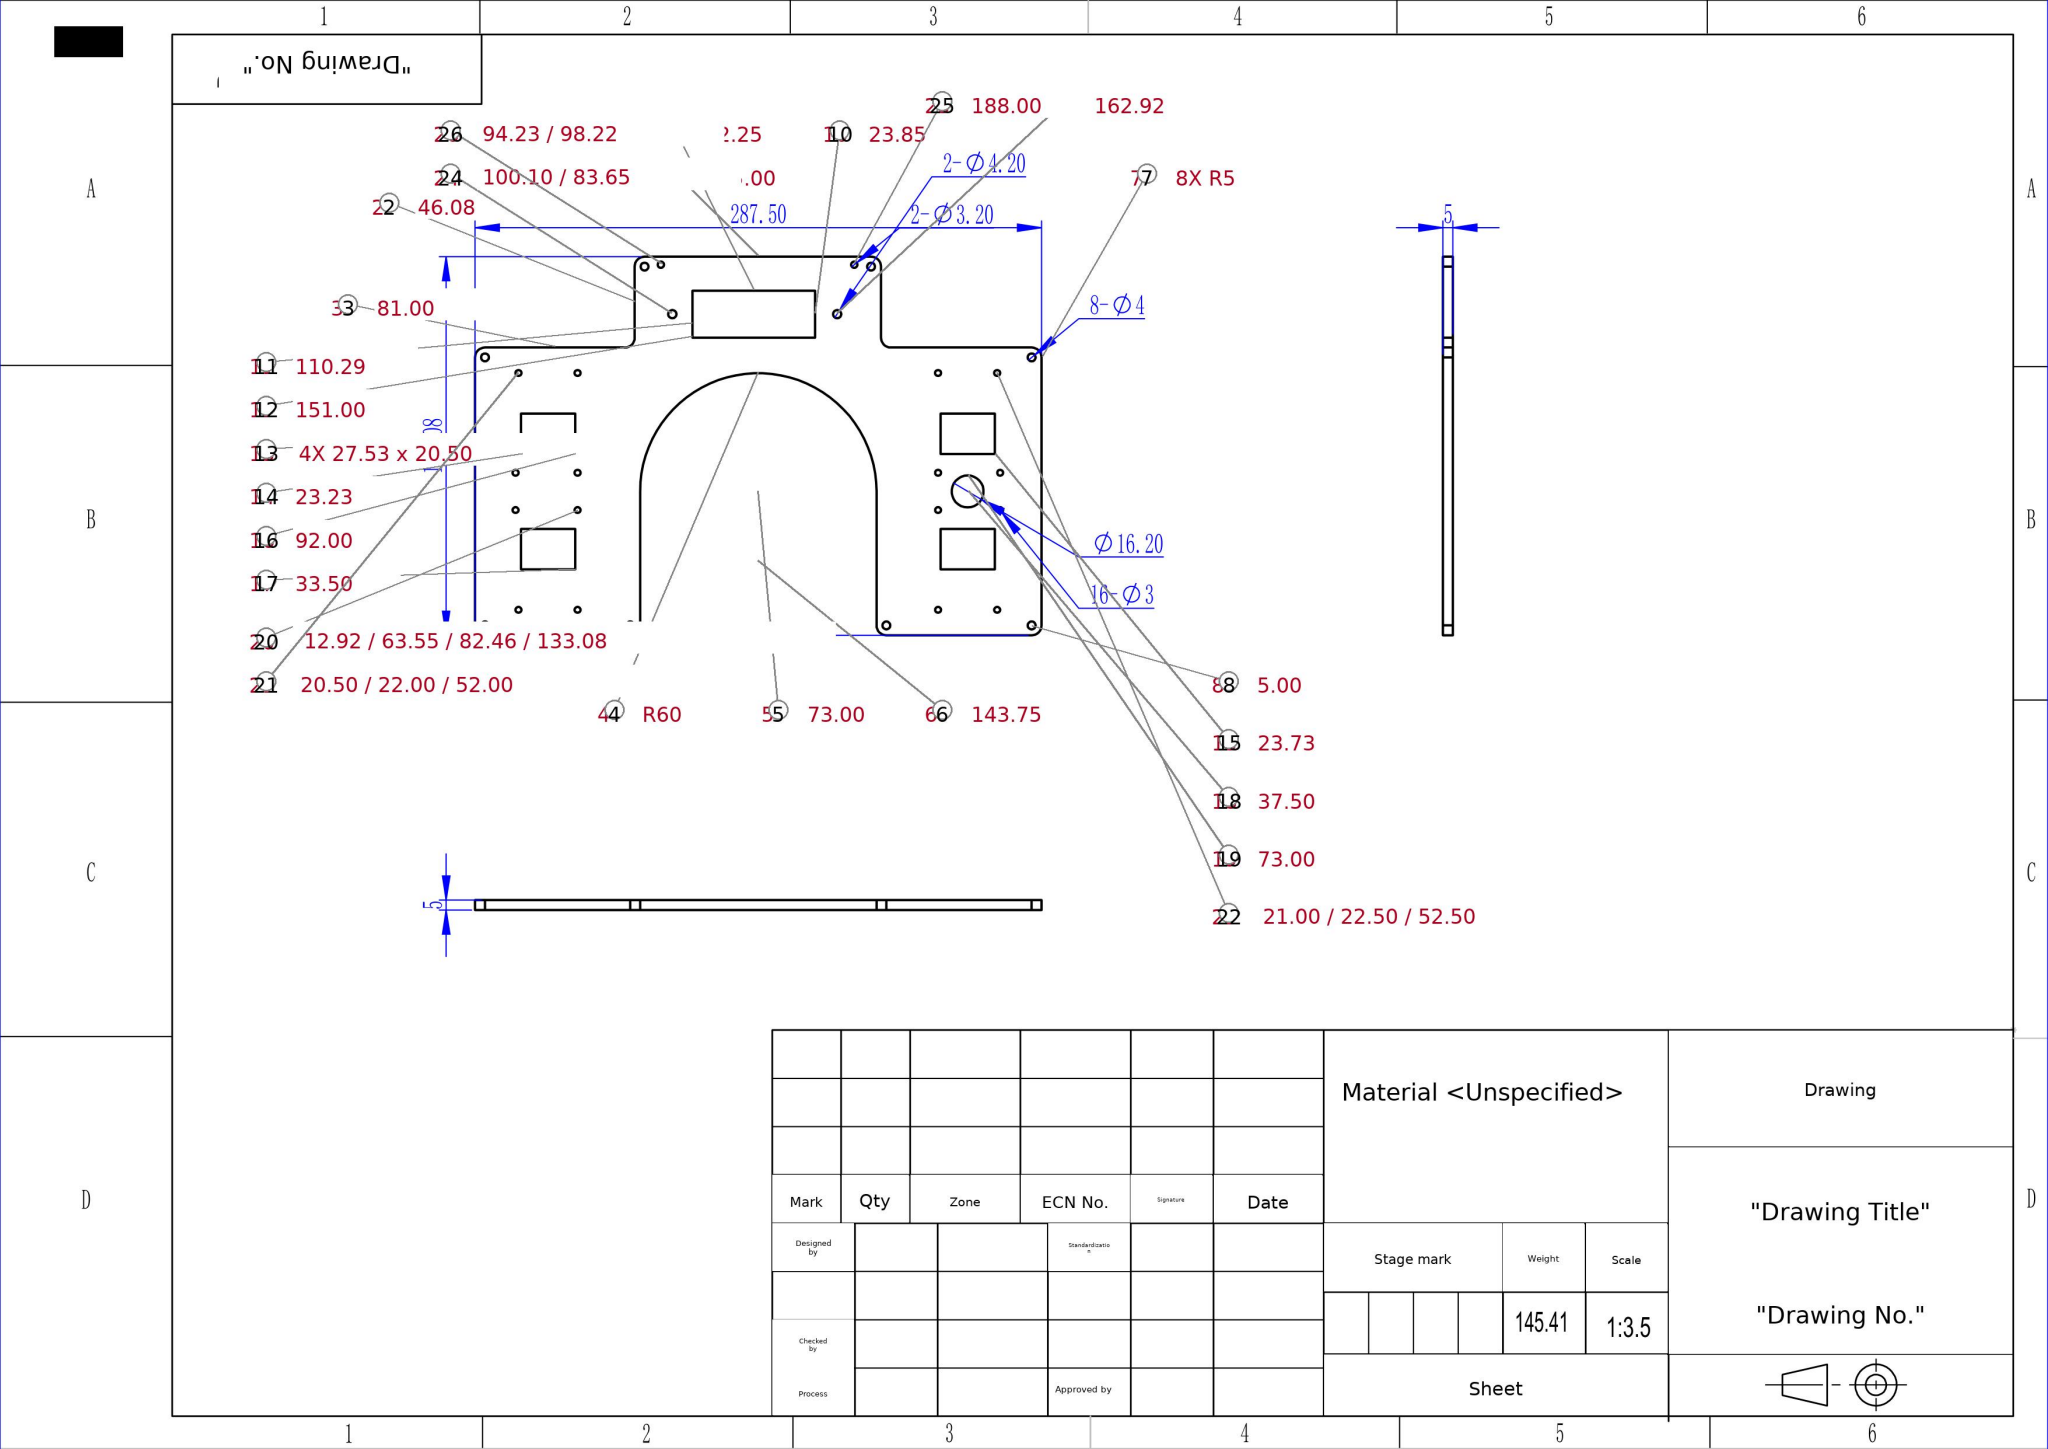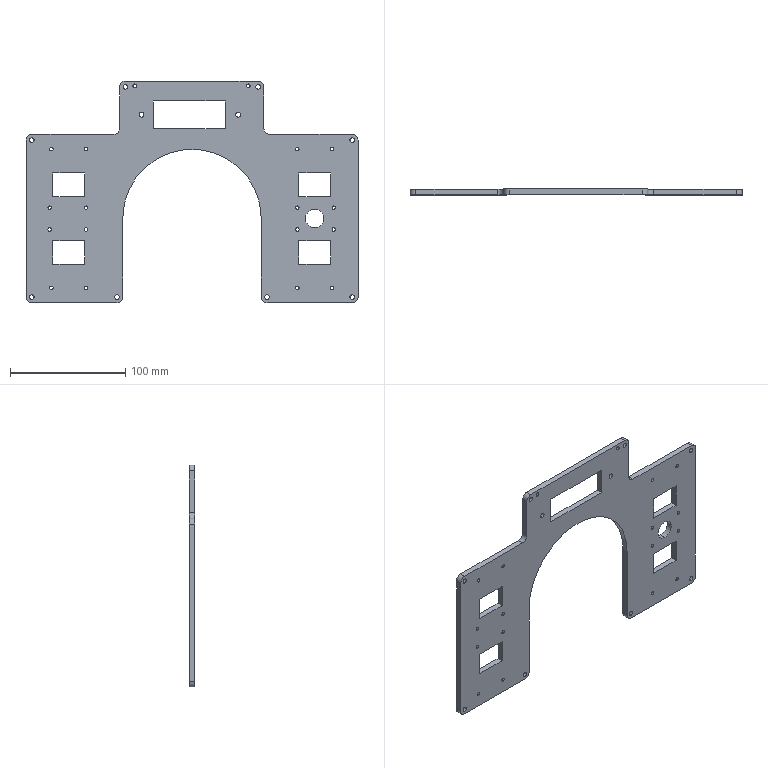Part | SolidWorks | mm | 1 solid | 102 faces | box 287.5 x 5 x 192.08 mm | volume 145408 mm3 | cylinder 69 | plane 33 | commonest cylinder face diameters 3 x32 4 x16 10 x10 4.2 x4 3.2 x4 16.2 x2 120 x1
build123d program:
from build123d import *

# Parameters (mm, degrees)
SKETCH1_R           = 2
SKETCH1_R_2         = 1.6
SKETCH1_R_3         = 8.1
SKETCH1_R_4         = 1.5
SKETCH1_R_5         = 2.1
SKETCH1_W           = 27.533
SKETCH1_H           = 20.5
SKETCH1_W_2         = 62.249
SKETCH1_H_2         = 23.847
BOSS_EXTRUDE1_DEPTH = 5


with BuildPart() as part:
    # Sketch1 → Boss-Extrude1 (new body)
    with BuildSketch(Plane(origin=(0, 0, 0), x_dir=(1, 0, 0), z_dir=(0, 1, 0))):
        with BuildLine():
            Line((-246.729, 44.894), (-246.729, -23.106))
            ThreePointArc((-246.729, -23.106), (-245.264, -26.642), (-241.729, -28.106))
            Line((-241.729, -28.106), (-170.729, -28.106))
            ThreePointArc((-170.729, -28.106), (-167.193, -29.571), (-165.729, -33.106))
            Line((-165.729, -33.106), (-165.729, -69.184))
            ThreePointArc((-165.729, -69.184), (-164.264, -72.72), (-160.729, -74.184))
            Line((-160.729, -74.184), (-45.729, -74.184))
            ThreePointArc((-45.729, -74.184), (-42.193, -72.72), (-40.729, -69.184))
            Line((-40.729, -69.184), (-40.729, -33.106))
            ThreePointArc((-40.729, -33.106), (-39.264, -29.571), (-35.729, -28.106))
            Line((-35.729, -28.106), (35.769, -28.106))
            ThreePointArc((35.769, -28.106), (39.305, -26.642), (40.769, -23.106))
            Line((40.769, -23.106), (40.769, 44.894))
            Line((40.769, 44.894), (40.769, 112.894))
            ThreePointArc((40.769, 112.894), (39.305, 116.429), (35.769, 117.894))
            Line((35.769, 117.894), (-37.98, 117.894))
            ThreePointArc((-37.98, 117.894), (-41.515, 116.429), (-42.98, 112.894))
            Line((-42.98, 112.894), (-42.98, 44.894))
            ThreePointArc((-42.98, 44.894), (-102.98, -15.106), (-162.98, 44.894))
            Line((-162.98, 44.894), (-162.98, 112.894))
            ThreePointArc((-162.98, 112.894), (-164.444, 116.429), (-167.98, 117.894))
            Line((-167.98, 117.894), (-241.729, 117.894))
            ThreePointArc((-241.729, 117.894), (-245.264, 116.429), (-246.729, 112.894))
            Line((-246.729, 112.894), (-246.729, 44.894))
        make_face()
        with Locations(Location((-160.729, -69.184, 0), (0, 0, 270))):
            Circle(SKETCH1_R, mode=Mode.SUBTRACT)
        with Locations(Location((-45.729, -69.184, 0), (0, 0, 270))):
            Circle(SKETCH1_R, mode=Mode.SUBTRACT)
        with Locations(Location((-241.729, -23.106, 0), (0, 0, 270))):
            Circle(SKETCH1_R, mode=Mode.SUBTRACT)
        with Locations(Location((35.769, -23.106, 0), (0, 0, 270))):
            Circle(SKETCH1_R, mode=Mode.SUBTRACT)
        with Locations(Location((-241.729, 112.894, 0), (0, 0, 270))):
            Circle(SKETCH1_R, mode=Mode.SUBTRACT)
        with Locations(Location((35.769, 112.894, 0), (0, 0, 270))):
            Circle(SKETCH1_R, mode=Mode.SUBTRACT)
        with Locations(Location((-167.98, 112.894, 0), (0, 0, 270))):
            Circle(SKETCH1_R, mode=Mode.SUBTRACT)
        with Locations(Location((-37.98, 112.894, 0), (0, 0, 270))):
            Circle(SKETCH1_R, mode=Mode.SUBTRACT)
        with Locations(Location((-152.499, -70.106, 0), (0, 0, 270))):
            Circle(SKETCH1_R_2, mode=Mode.SUBTRACT)
        with Locations(Location((-54.279, -70.106, 0), (0, 0, 270))):
            Circle(SKETCH1_R_2, mode=Mode.SUBTRACT)
        with Locations(Location((3.273, 44.894, 0), (0, 0, 270))):
            Circle(SKETCH1_R_3, mode=Mode.SUBTRACT)
        with Locations(Location((-224.729, -15.184, 0), (0, 0, 270))):
            Circle(SKETCH1_R_4, mode=Mode.SUBTRACT)
        with Locations(Location((-194.727, -15.184, 0), (0, 0, 270))):
            Circle(SKETCH1_R_4, mode=Mode.SUBTRACT)
        with Locations(Location((-226.229, 35.438, 0), (0, 0, 270))):
            Circle(SKETCH1_R_4, mode=Mode.SUBTRACT)
        with Locations(Location((-194.727, 35.438, 0), (0, 0, 270))):
            Circle(SKETCH1_R_4, mode=Mode.SUBTRACT)
        with Locations(Location((-194.727, 104.972, 0), (0, 0, 90))):
            Circle(SKETCH1_R_4, mode=Mode.SUBTRACT)
        with Locations(Location((-224.729, 104.972, 0), (0, 0, 90))):
            Circle(SKETCH1_R_4, mode=Mode.SUBTRACT)
        with Locations(Location((-226.229, 54.349, 0), (0, 0, 90))):
            Circle(SKETCH1_R_4, mode=Mode.SUBTRACT)
        with Locations(Location((-194.727, 54.349, 0), (0, 0, 90))):
            Circle(SKETCH1_R_4, mode=Mode.SUBTRACT)
        with Locations(Location((-11.729, -15.186, 0), (0, 0, 90))):
            Circle(SKETCH1_R_4, mode=Mode.SUBTRACT)
        with Locations(Location((18.272, -15.186, 0), (0, 0, 90))):
            Circle(SKETCH1_R_4, mode=Mode.SUBTRACT)
        with Locations(Location((-11.729, 35.437, 0), (0, 0, 90))):
            Circle(SKETCH1_R_4, mode=Mode.SUBTRACT)
        with Locations(Location((19.773, 35.436, 0), (0, 0, 90))):
            Circle(SKETCH1_R_4, mode=Mode.SUBTRACT)
        with Locations(Location((-11.728, 54.348, 0), (0, 0, 270))):
            Circle(SKETCH1_R_4, mode=Mode.SUBTRACT)
        with Locations(Location((19.773, 54.348, 0), (0, 0, 270))):
            Circle(SKETCH1_R_4, mode=Mode.SUBTRACT)
        with Locations(Location((-11.728, 104.971, 0), (0, 0, 270))):
            Circle(SKETCH1_R_4, mode=Mode.SUBTRACT)
        with Locations(Location((18.274, 104.97, 0), (0, 0, 270))):
            Circle(SKETCH1_R_4, mode=Mode.SUBTRACT)
        with Locations(Location((-146.633, -45.03, 0), (0, 0, 270))):
            Circle(SKETCH1_R_5, mode=Mode.SUBTRACT)
        with Locations(Location((-62.98, -45.03, 0), (0, 0, 270))):
            Circle(SKETCH1_R_5, mode=Mode.SUBTRACT)
        with Locations((-209.729, 74.144)):
            Rectangle(SKETCH1_W, SKETCH1_H, mode=Mode.SUBTRACT)
        with Locations((-209.729, 15.644)):
            Rectangle(SKETCH1_W, SKETCH1_H, mode=Mode.SUBTRACT)
        Polygon((-10.494, 5.392), (-10.494, 25.892), (17.039, 25.892), (17.039, 5.392), align=None, mode=Mode.SUBTRACT)
        Polygon((17.04, 63.892), (-10.493, 63.892), (-10.493, 84.392), (17.04, 84.392), align=None, mode=Mode.SUBTRACT)
        with Locations((-105.317, -45.03)):
            Rectangle(SKETCH1_W_2, SKETCH1_H_2, mode=Mode.SUBTRACT)
    extrude(amount=BOSS_EXTRUDE1_DEPTH)


solid = part.part